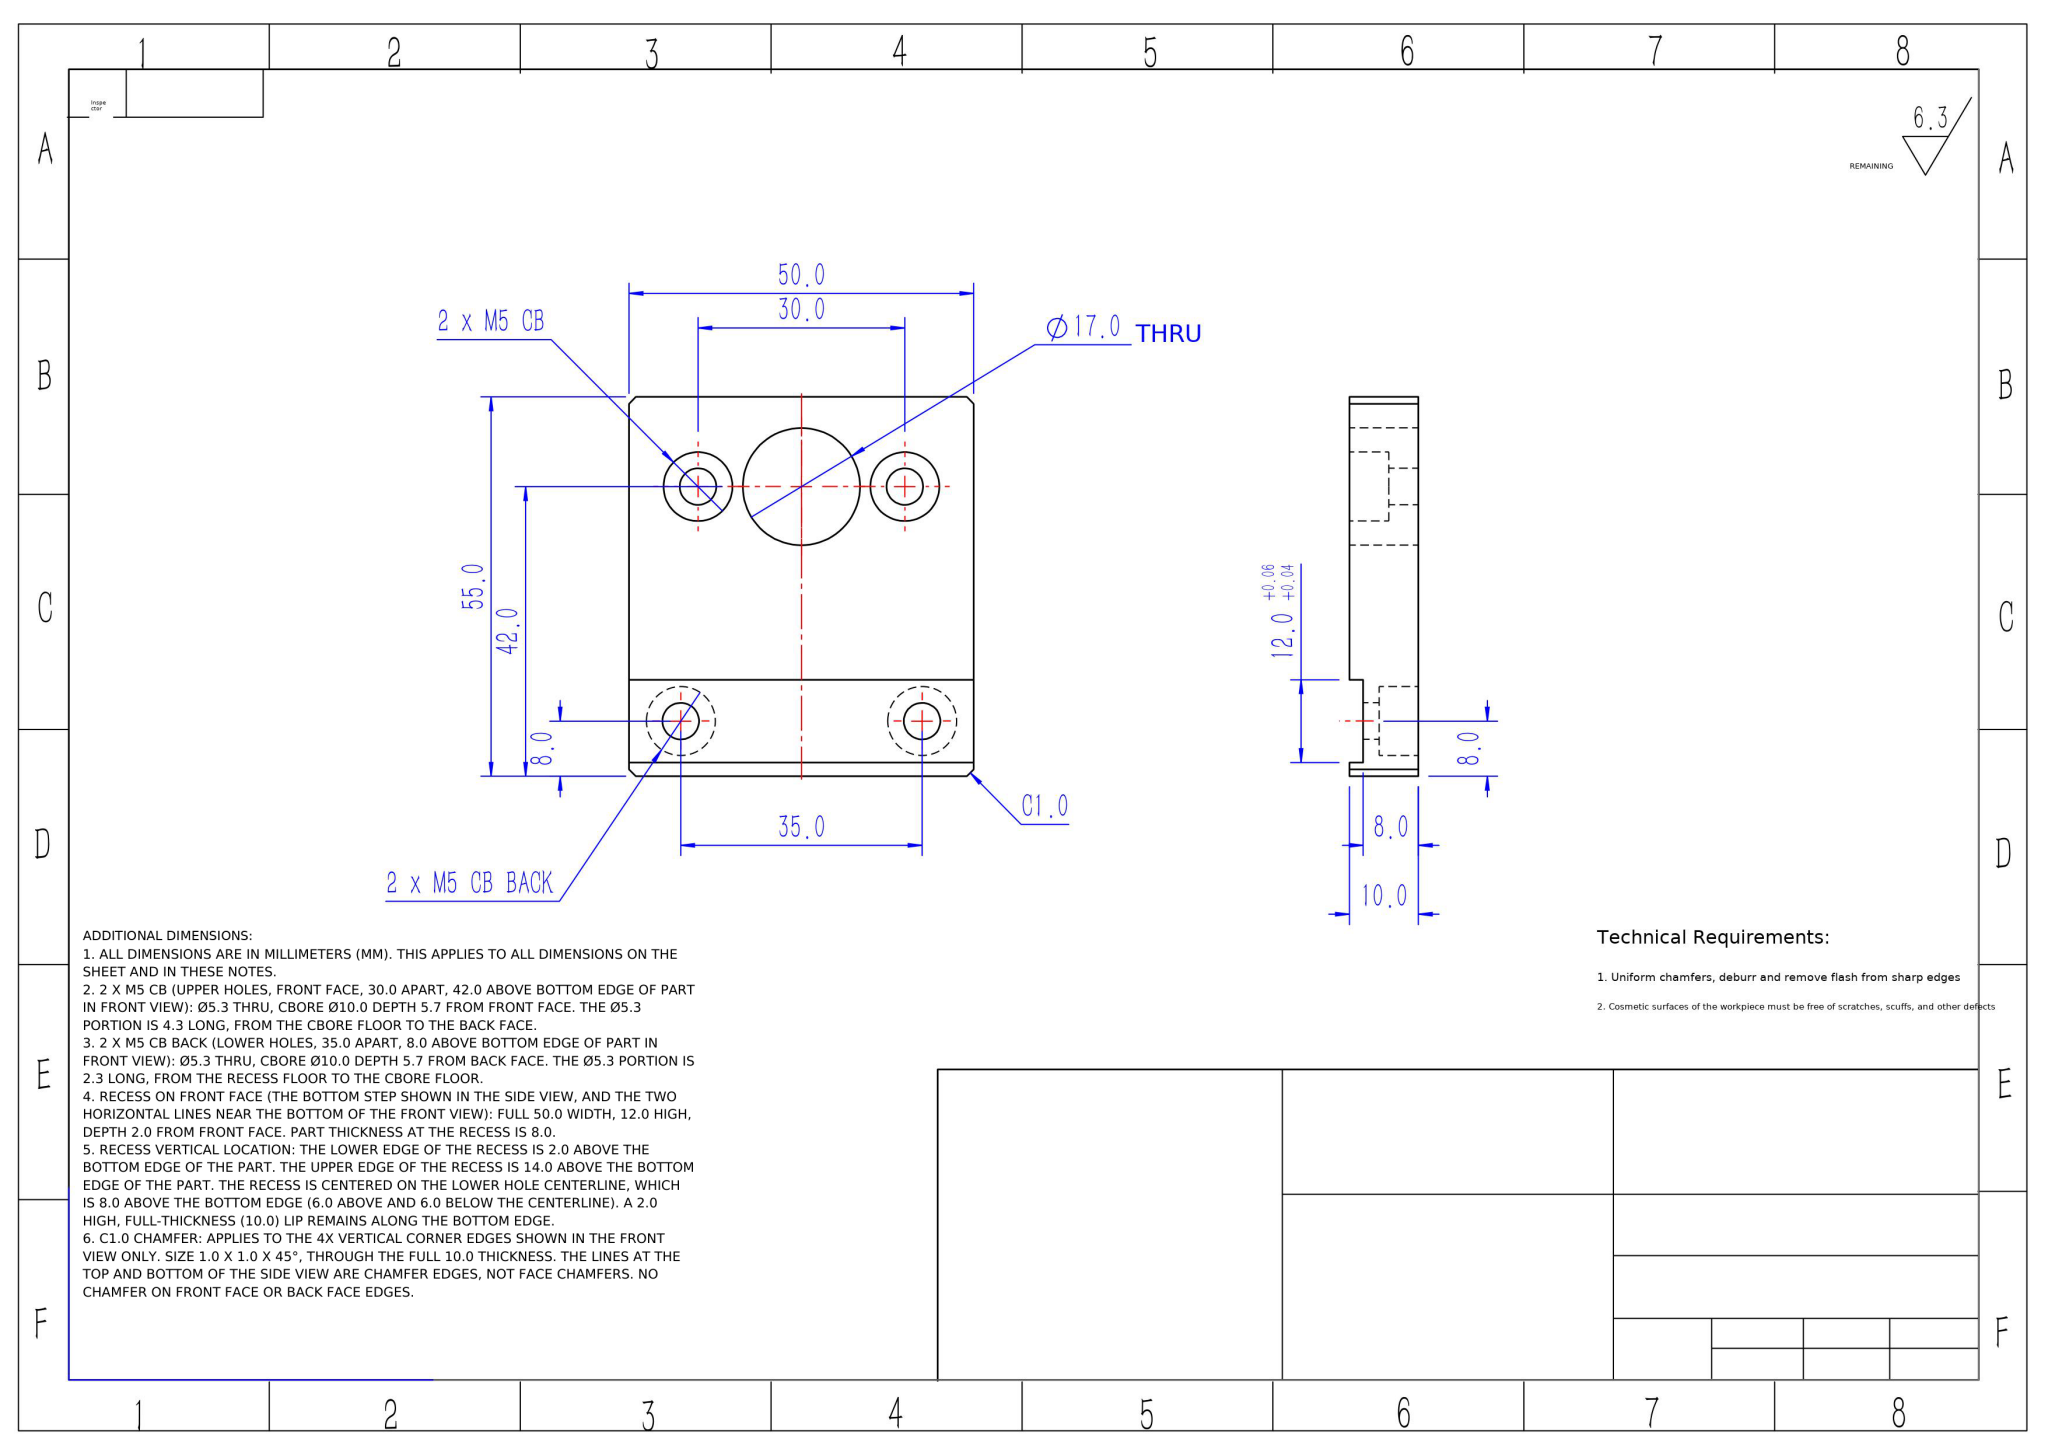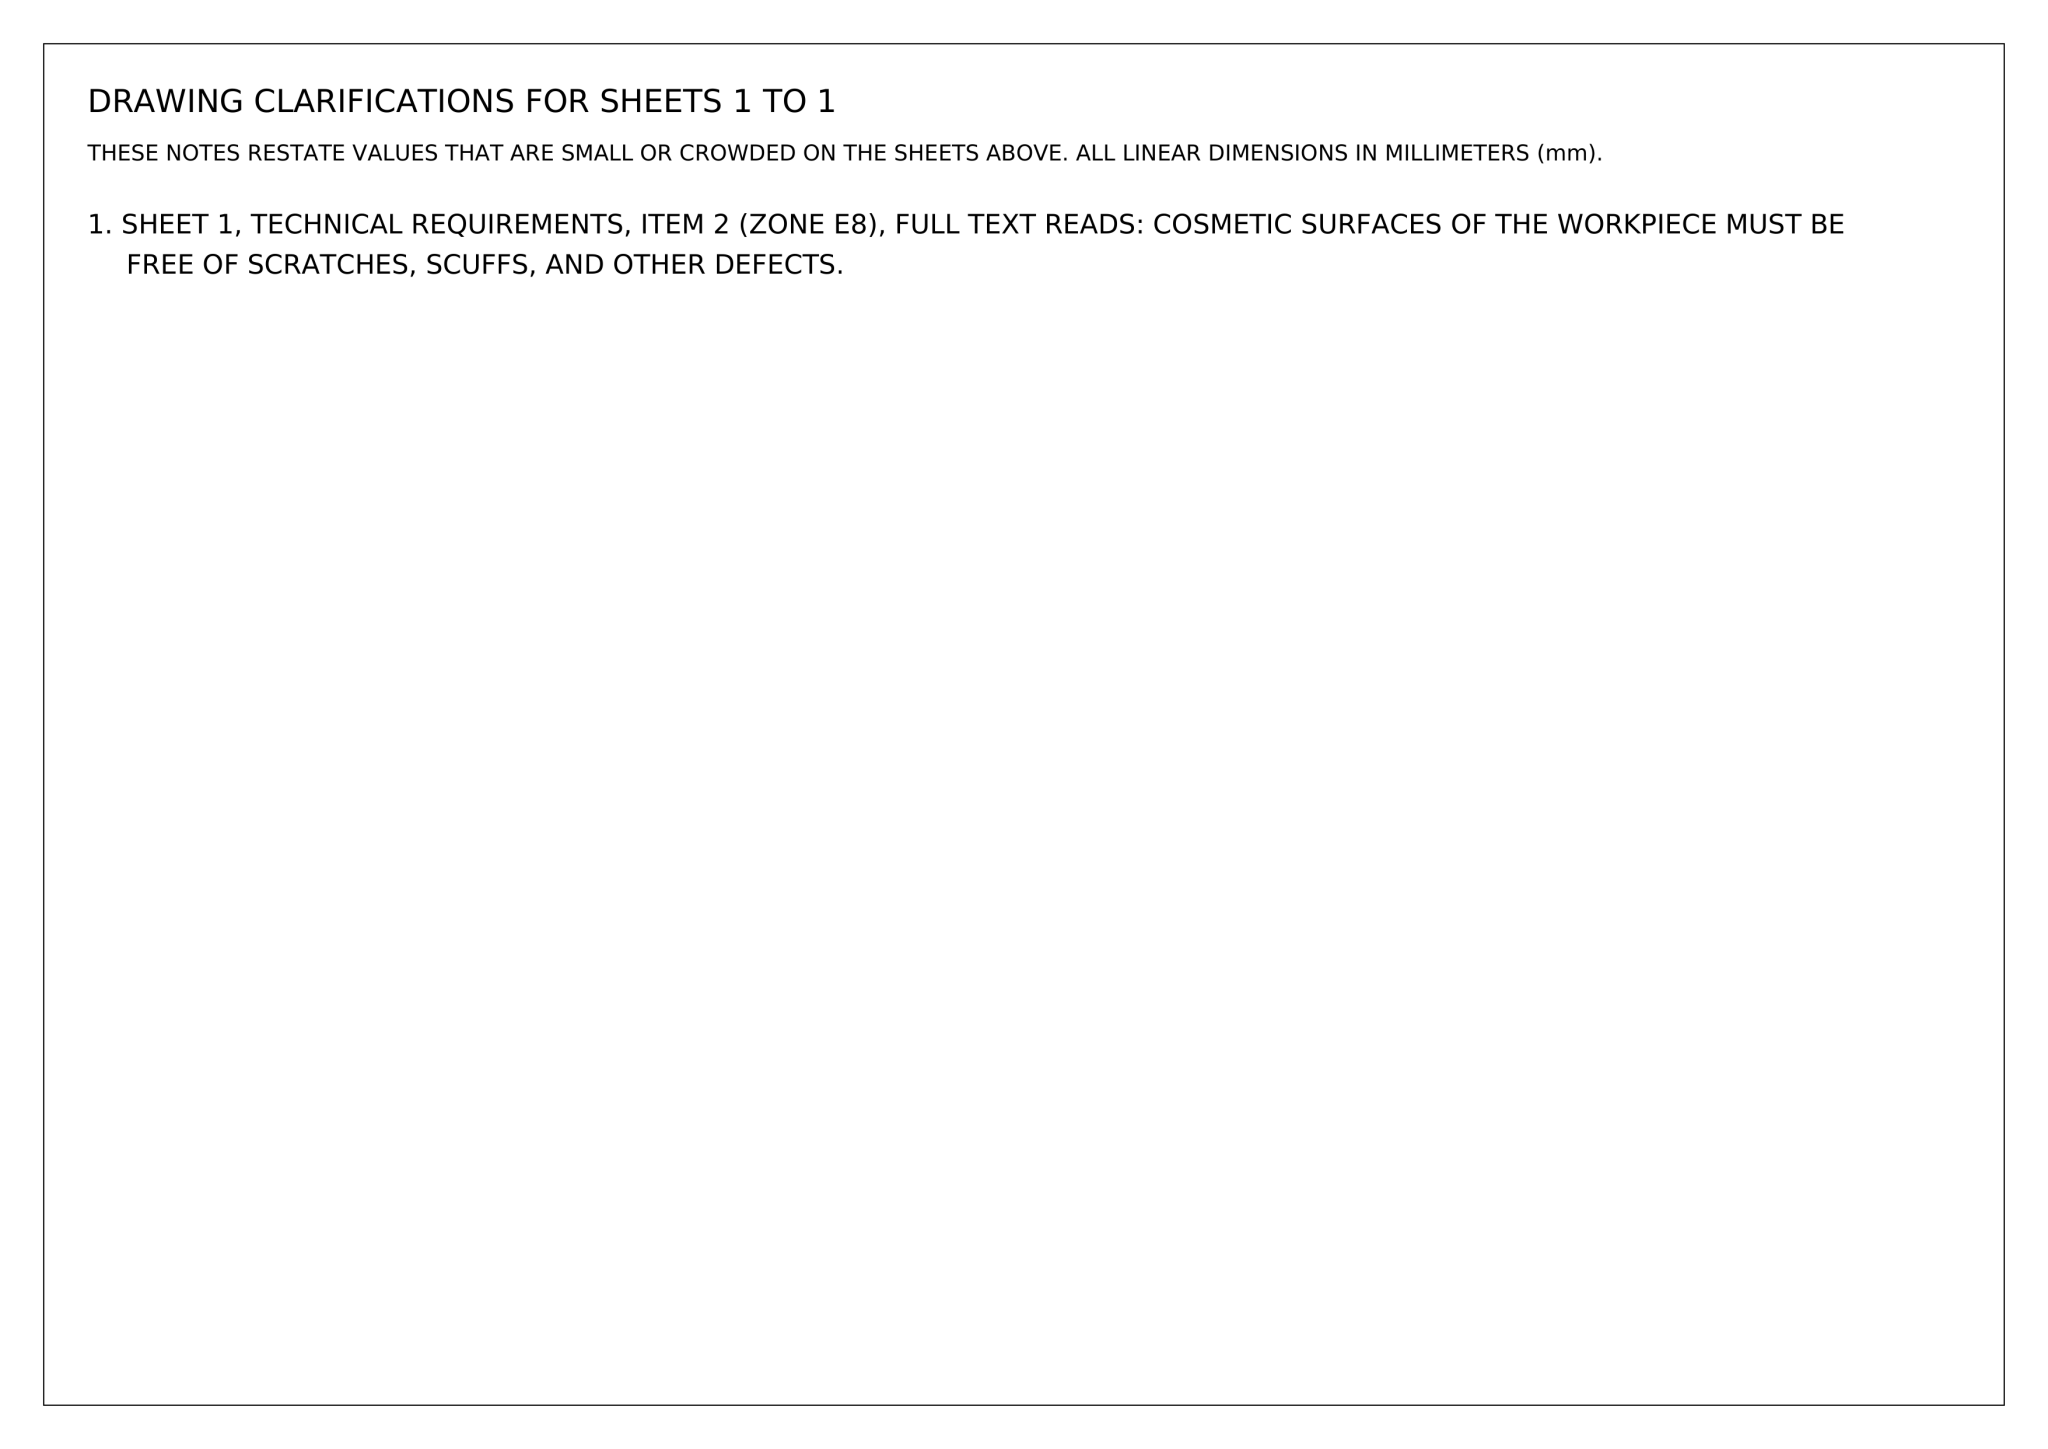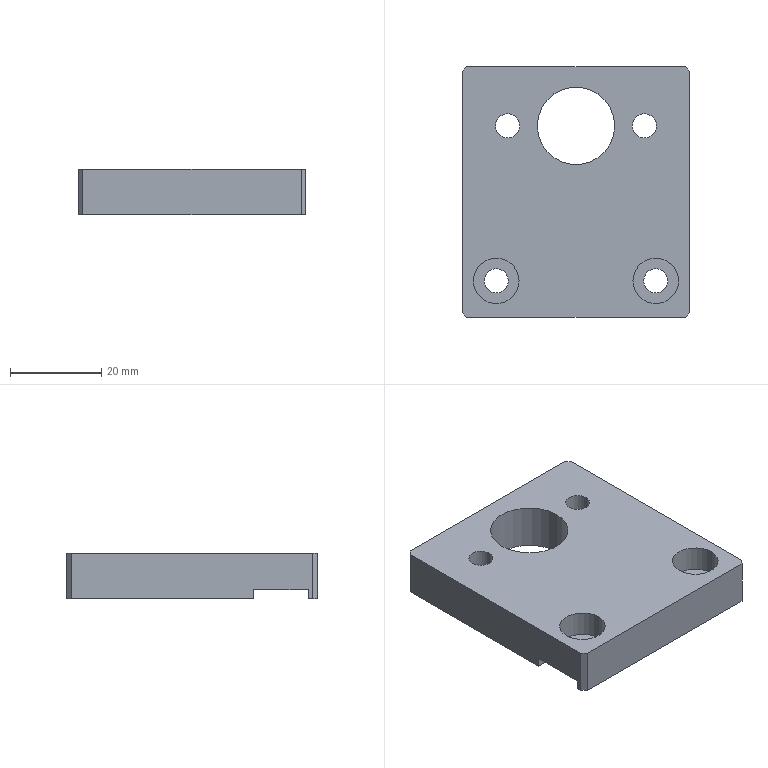Part | NX | mm | 1 solid | 36 faces | box 50 x 55 x 10 mm | volume 21928 mm3 | cylinder 18 | plane 18 | commonest cylinder face diameters 10 x8 5.3 x8 17 x2